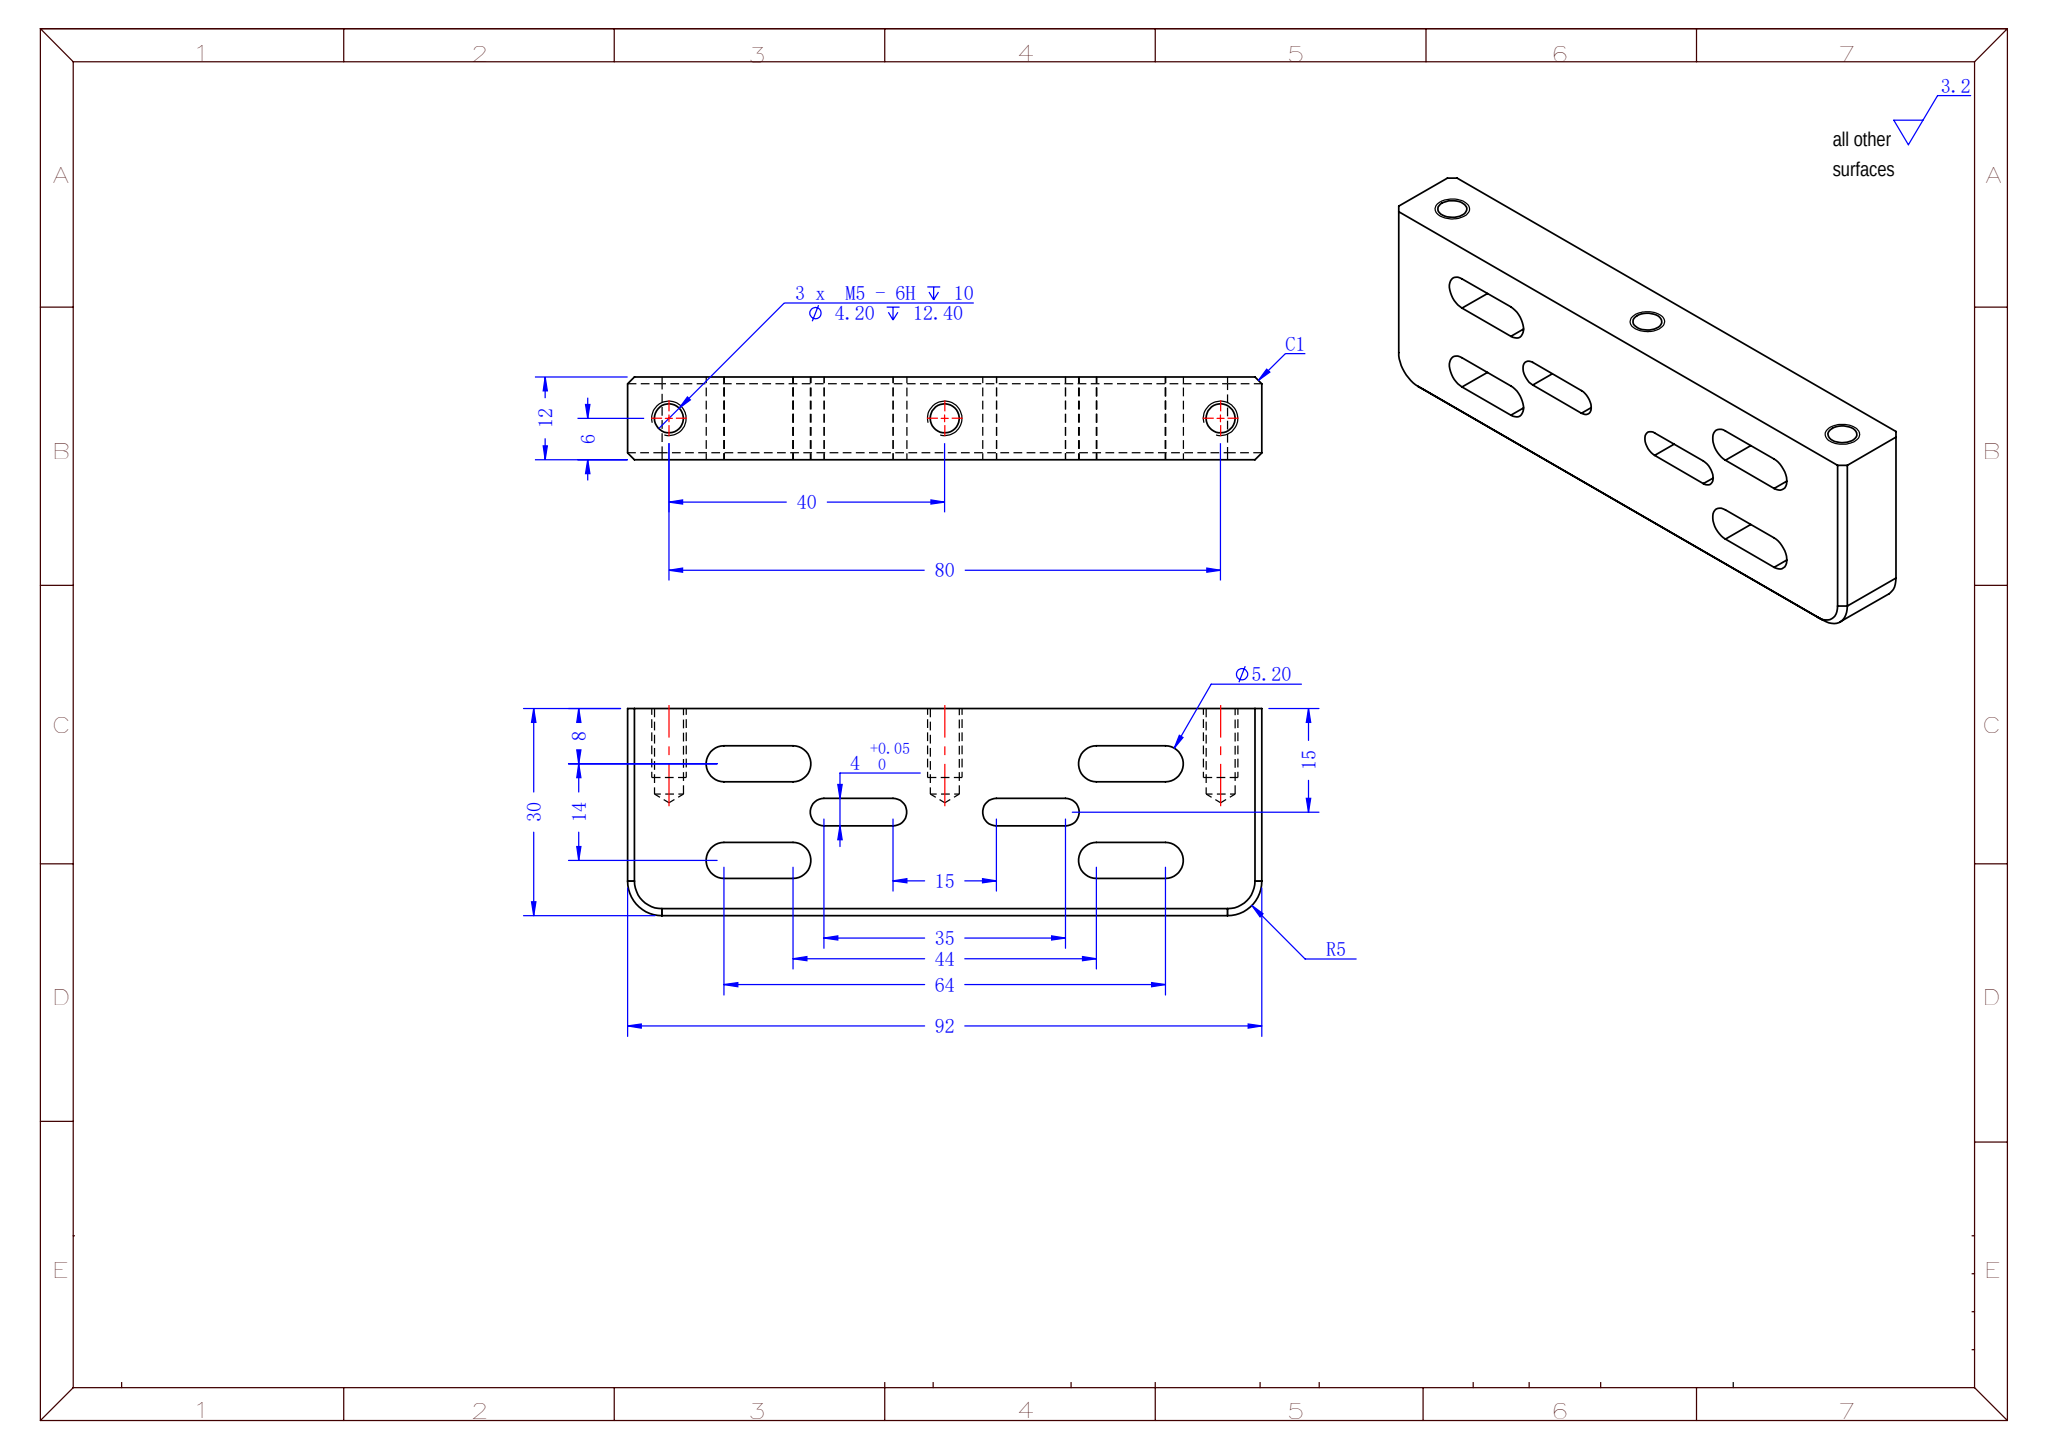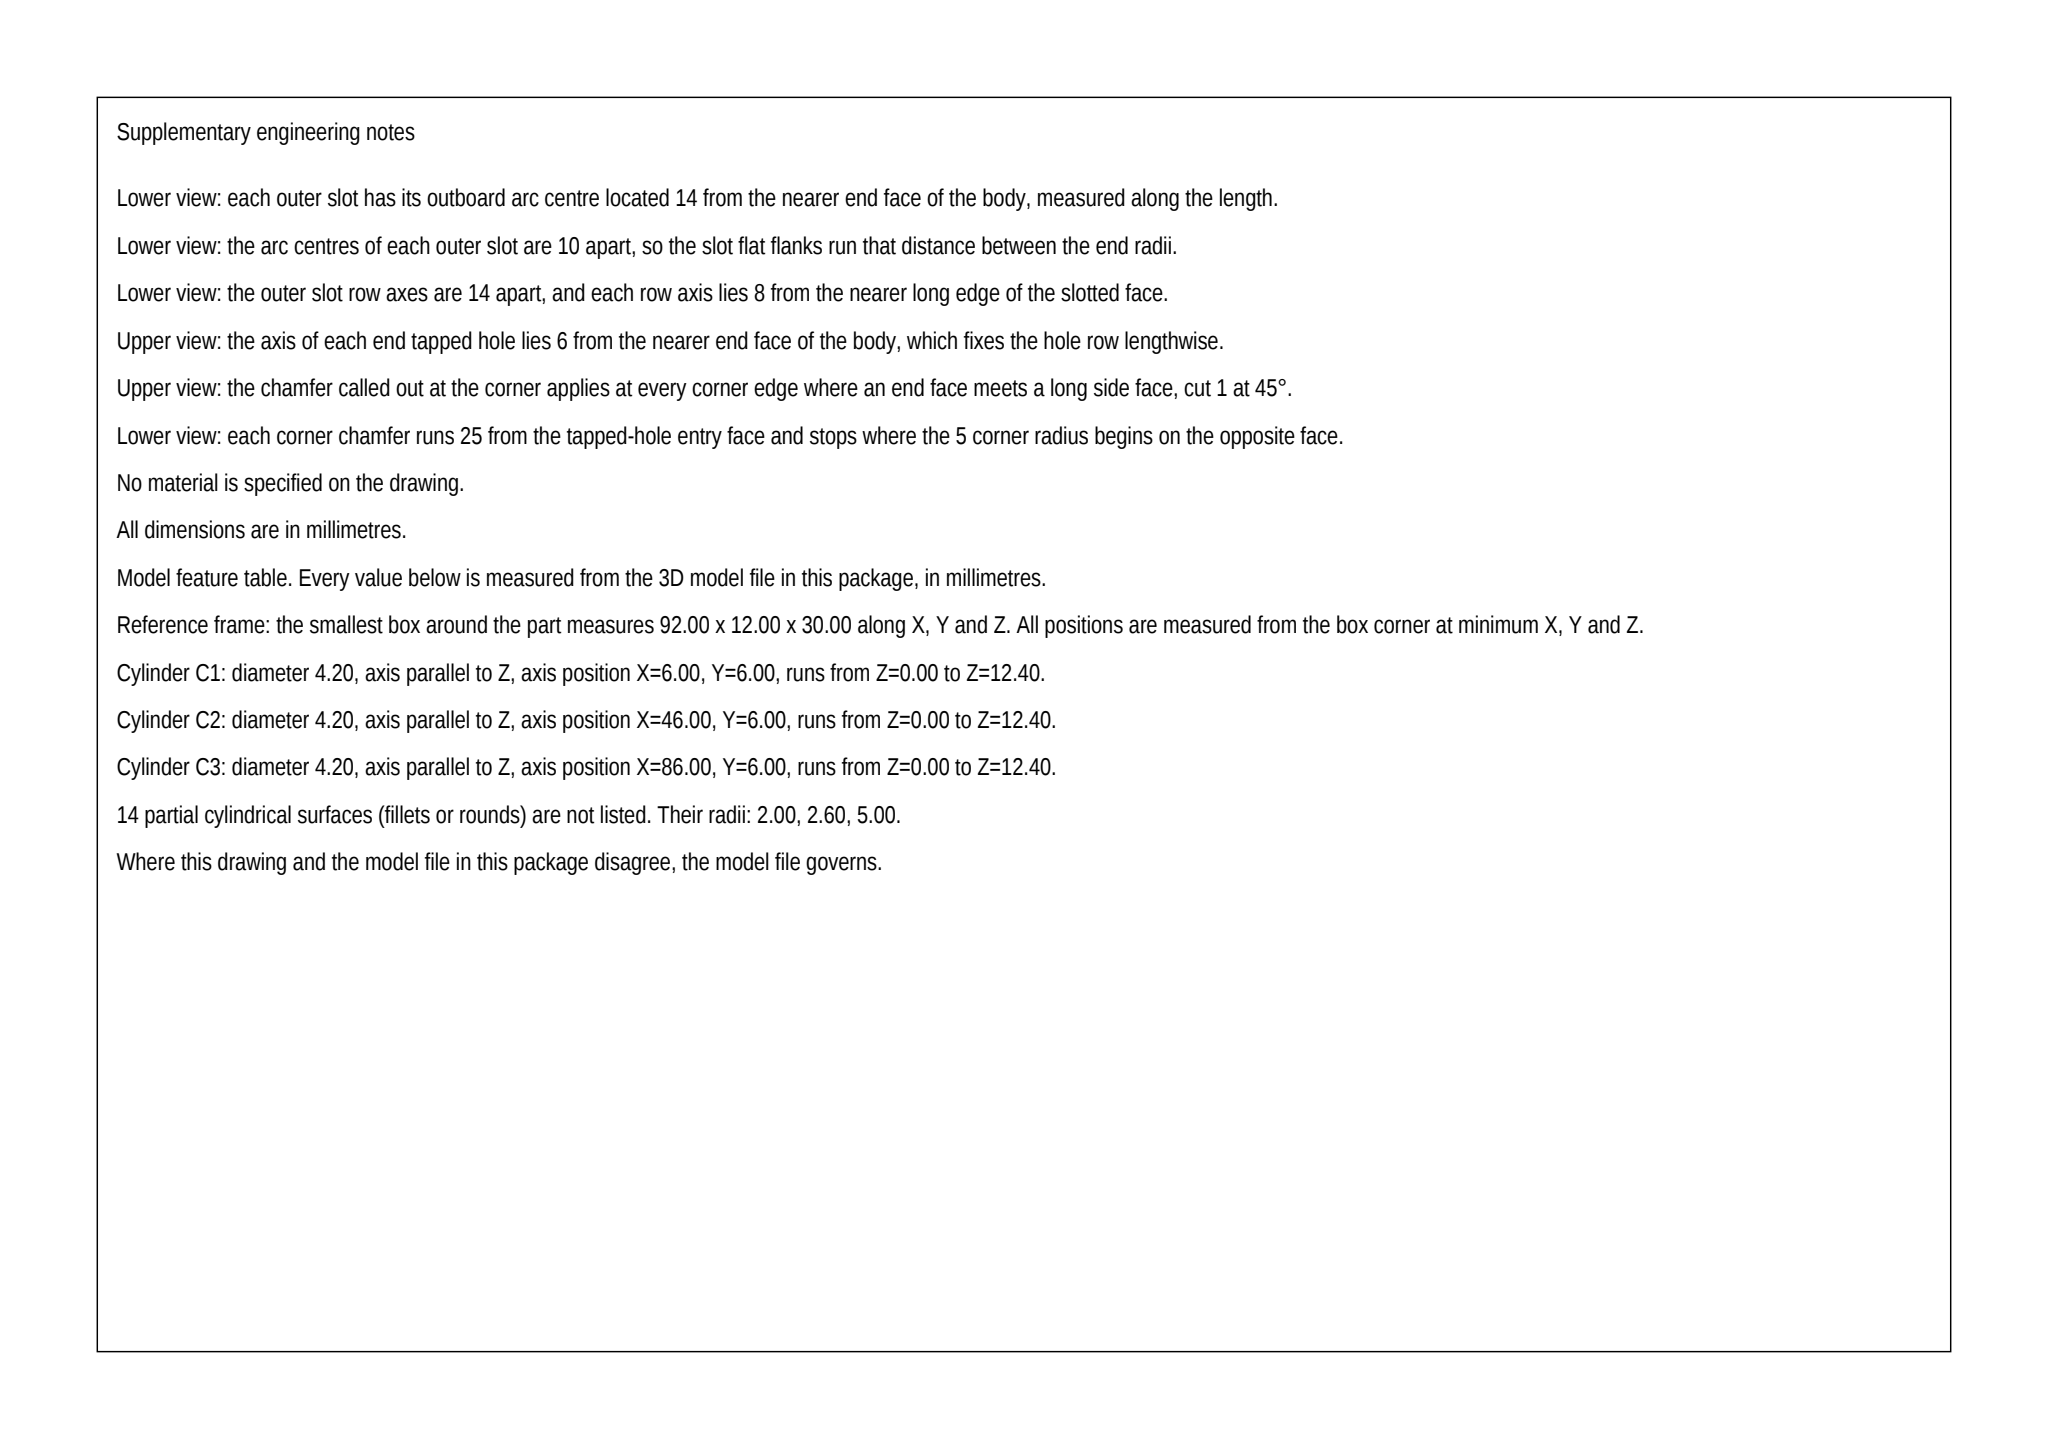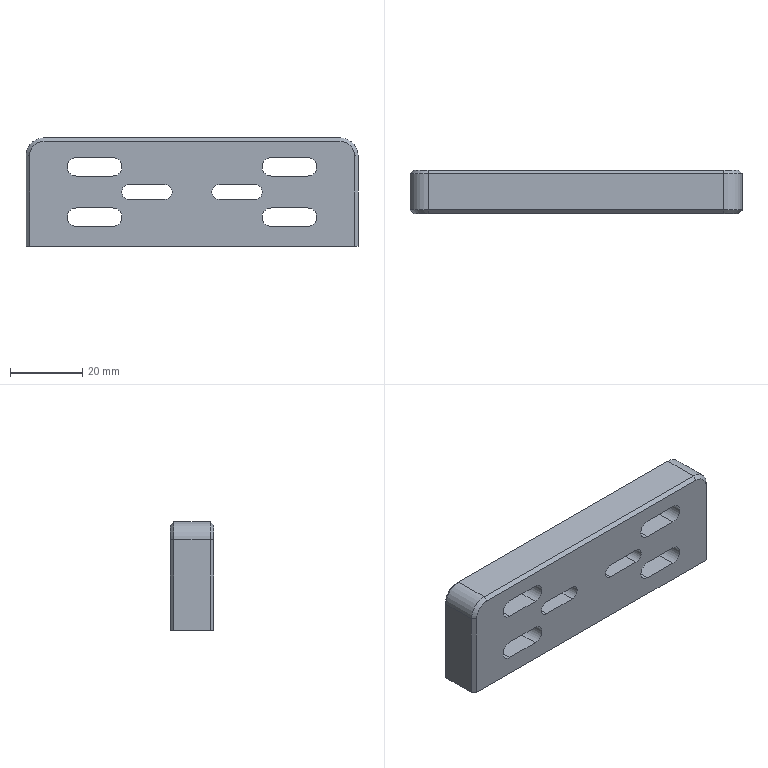Part | SolidWorks | mm | 1 solid | 54 faces | box 92 x 12 x 30 mm | volume 27535 mm3 | plane 24 | cylinder 20 | cone 10 | commonest cylinder face diameters 5.2 x8 4.2 x6 4 x4 10 x2
Drawing notes:
MATL THK 12 TYP BOTH LEGS | from the solid: Planes y=0 and y=12; all slot cyls axis y, length 12 = through thk
4X Ø5.20 SLOT THRU: 15.20 OAL, 10 C-C | from the solid: Ø5.2 y-axis cyl pairs x=14/24 and x=68/78 at z=8 & 22, len 12: 10 C-C +5.2
2X 4 +0.05/0 SLOT THRU: 14 OAL, 10 C-C | from the solid: Ø4.0 y-axis cyl pairs x=28.5/38.5 and x=53.5/63.5 at z=15, len 12: 10 C-C +4
SLOT CL 8, 15 & 22 UP FROM BTM EDGE | from the solid: Ø5.2 cyls at z=8 and z=22; Ø4.0 cyls at z=15; bbox z 0-30
SLOT END CL FROM LH EDGE: 14, 24, 68, 78 (Ø5.20); 28.5, 38.5, 53.5, 63.5 (4 WIDE) | from the solid: Ø5.2 cyls x=14,24,68,78; Ø4.0 cyls x=28.5,38.5,53.5,63.5; bbox x 0-92
2X Ø10 x 10 DP, CL 25 UP, 5 & 87 FROM LH EDGE | from the solid: Ø10 y-axis cyls at [5,null,25] and [87,null,25], length 10
4X CSK Ø8 X 90°, BOTH ENDS OF 2X 4 WIDE SLOTS ON 15 CL | from the solid: cones[90.0, ref_dia 8.0] qty 4 at ends of Ø4 y-axis slots at x=28.5/38.5 and 53.5/63.5, z=15
build123d program:
from build123d import *

# Parameters (mm, degrees)
SKETCH1_W             = 92
SKETCH1_H             = 30
BOSS_EXTRUDE1_DEPTH   = 6
M5_TAPPED_HOLE1_D     = 4.2
M5_TAPPED_HOLE1_DEPTH = 12.4
M5_TAPPED_HOLE1_TIP   = 1.262
CUT_EXTRUDE1_DEPTH    = 50.85
CUT_EXTRUDE2_DEPTH    = 50.85
FILLET1_R             = 5
CHAMFER1_SIZE         = 1


with BuildPart() as part:
    # Sketch1 → Boss-Extrude1 (new, symmetric)
    with BuildSketch(Plane(origin=(0, 0, 0), x_dir=(1, 0, 0), z_dir=(0, 1, 0))):
        Rectangle(SKETCH1_W, SKETCH1_H)
    extrude(amount=BOSS_EXTRUDE1_DEPTH, both=True)

    # M5 Tapped Hole1
    with Locations(Plane(origin=(0, 0, -15), x_dir=(-1, 0, 0), z_dir=(0, 0, -1))):
        with Locations((-40, 0), (0, 0), (40, 0)):
            Hole(M5_TAPPED_HOLE1_D / 2, depth=M5_TAPPED_HOLE1_DEPTH)
            with Locations((0, 0, -(M5_TAPPED_HOLE1_DEPTH + M5_TAPPED_HOLE1_TIP / 2))):  # 118° drill point
                Cone(0, M5_TAPPED_HOLE1_D / 2, M5_TAPPED_HOLE1_TIP, mode=Mode.SUBTRACT)

    # Sketch4 → Cut-Extrude1 (cut, through all)
    with BuildSketch(Plane(origin=(0, 6, 0), x_dir=(1, 0, 0), z_dir=(0, 1, 0))):
        with BuildLine():
            Line((-32, 9.6), (-22, 9.6))
            ThreePointArc((-22, 9.6), (-19.4, 7), (-22, 4.4))
            Line((-22, 4.4), (-32, 4.4))
            ThreePointArc((-32, 4.4), (-34.6, 7), (-32, 9.6))
        make_face()
        with BuildLine():
            Line((-32, -4.4), (-22, -4.4))
            ThreePointArc((-22, -4.4), (-19.4, -7), (-22, -9.6))
            Line((-22, -9.6), (-32, -9.6))
            ThreePointArc((-32, -9.6), (-34.6, -7), (-32, -4.4))
        make_face()
        with BuildLine():
            Line((22, 9.6), (32, 9.6))
            ThreePointArc((32, 9.6), (34.6, 7), (32, 4.4))
            Line((32, 4.4), (22, 4.4))
            ThreePointArc((22, 4.4), (19.4, 7), (22, 9.6))
        make_face()
        with BuildLine():
            Line((22, -4.4), (32, -4.4))
            ThreePointArc((32, -4.4), (34.6, -7), (32, -9.6))
            Line((32, -9.6), (22, -9.6))
            ThreePointArc((22, -9.6), (19.4, -7), (22, -4.4))
        make_face()
    extrude(amount=-CUT_EXTRUDE1_DEPTH, mode=Mode.SUBTRACT)

    # Sketch5 → Cut-Extrude2 (cut, through all)
    with BuildSketch(Plane(origin=(0, 6, 0), x_dir=(1, 0, 0), z_dir=(0, 1, 0))):
        with BuildLine():
            Line((7.5, 2), (17.5, 2))
            ThreePointArc((17.5, 2), (19.5, 0), (17.5, -2))
            Line((17.5, -2), (7.5, -2))
            ThreePointArc((7.5, -2), (5.5, 0), (7.5, 2))
        make_face()
        with BuildLine():
            Line((-17.5, 2), (-7.5, 2))
            ThreePointArc((-7.5, 2), (-5.5, 0), (-7.5, -2))
            Line((-7.5, -2), (-17.5, -2))
            ThreePointArc((-17.5, -2), (-19.5, 0), (-17.5, 2))
        make_face()
    extrude(amount=-CUT_EXTRUDE2_DEPTH, mode=Mode.SUBTRACT)

    # Fillet1
    fillet1_edges = [part.edges().sort_by_distance(p)[0] for p in [
        (46, 0, 15),
        (-46, 0, 15),
    ]]
    fillet(fillet1_edges, radius=FILLET1_R)

    # Chamfer1
    chamfer1_edges = [part.edges().sort_by_distance(p)[0] for p in [
        (-46, 6, -2.5),
        (0, -6, 15),
        (0, 6, 15),
        (46, -6, -2.5),
        (44.536, -6, 13.536),
        (-44.536, -6, 13.536),
        (46, 6, -2.5),
        (44.536, 6, 13.536),
        (-44.536, 6, 13.536),
        (-46, -6, -2.5),
    ]]
    chamfer(chamfer1_edges, length=CHAMFER1_SIZE)


solid = part.part